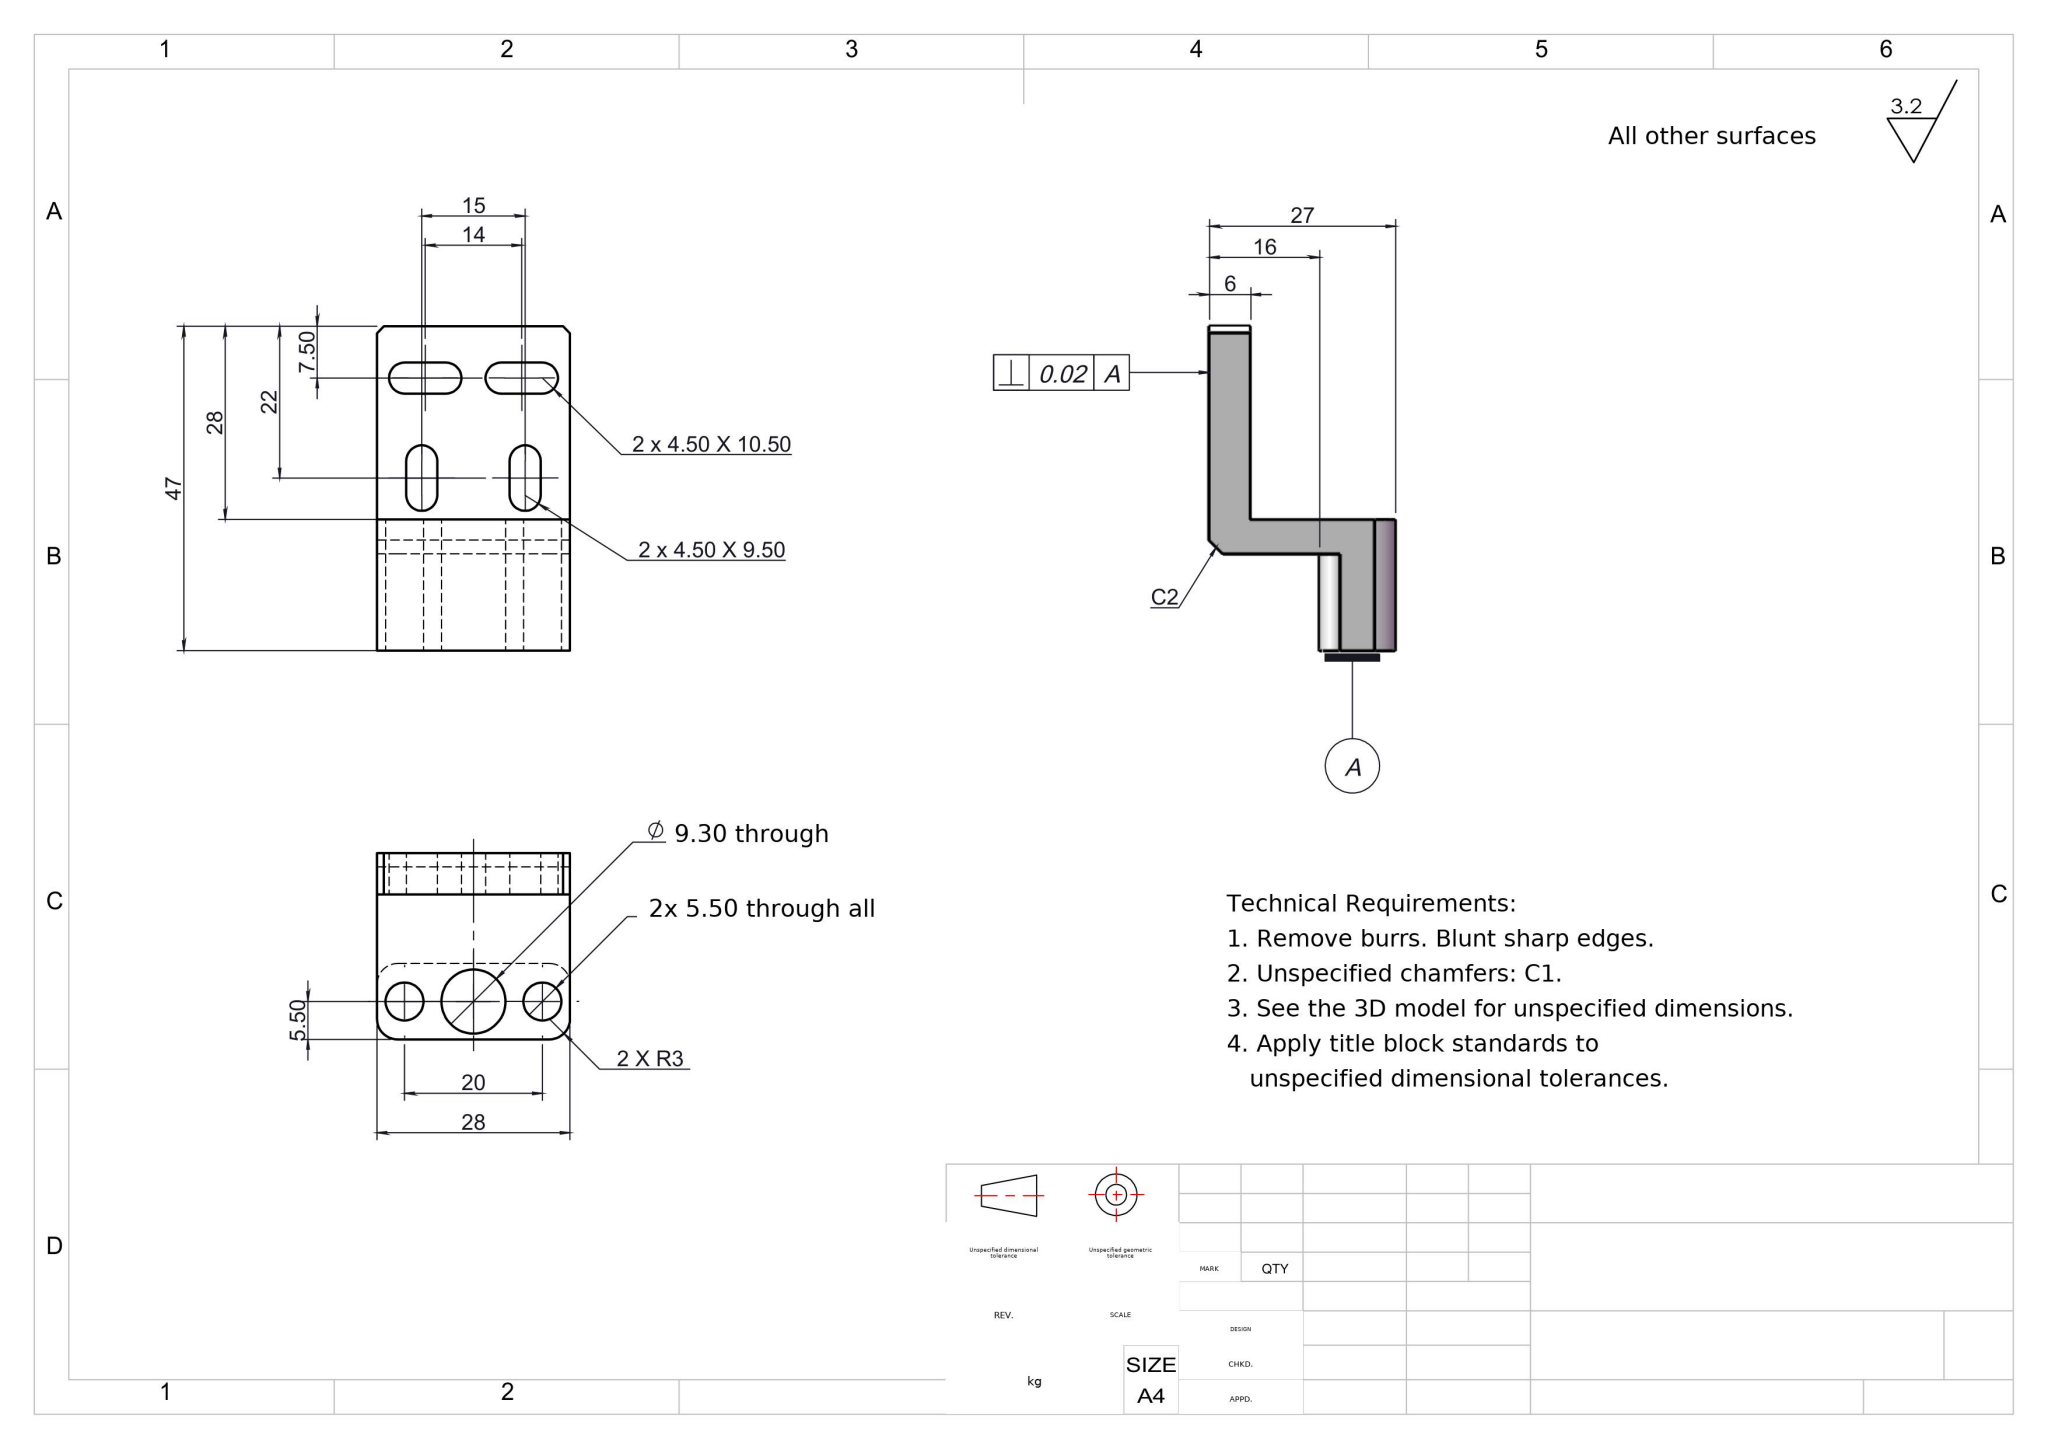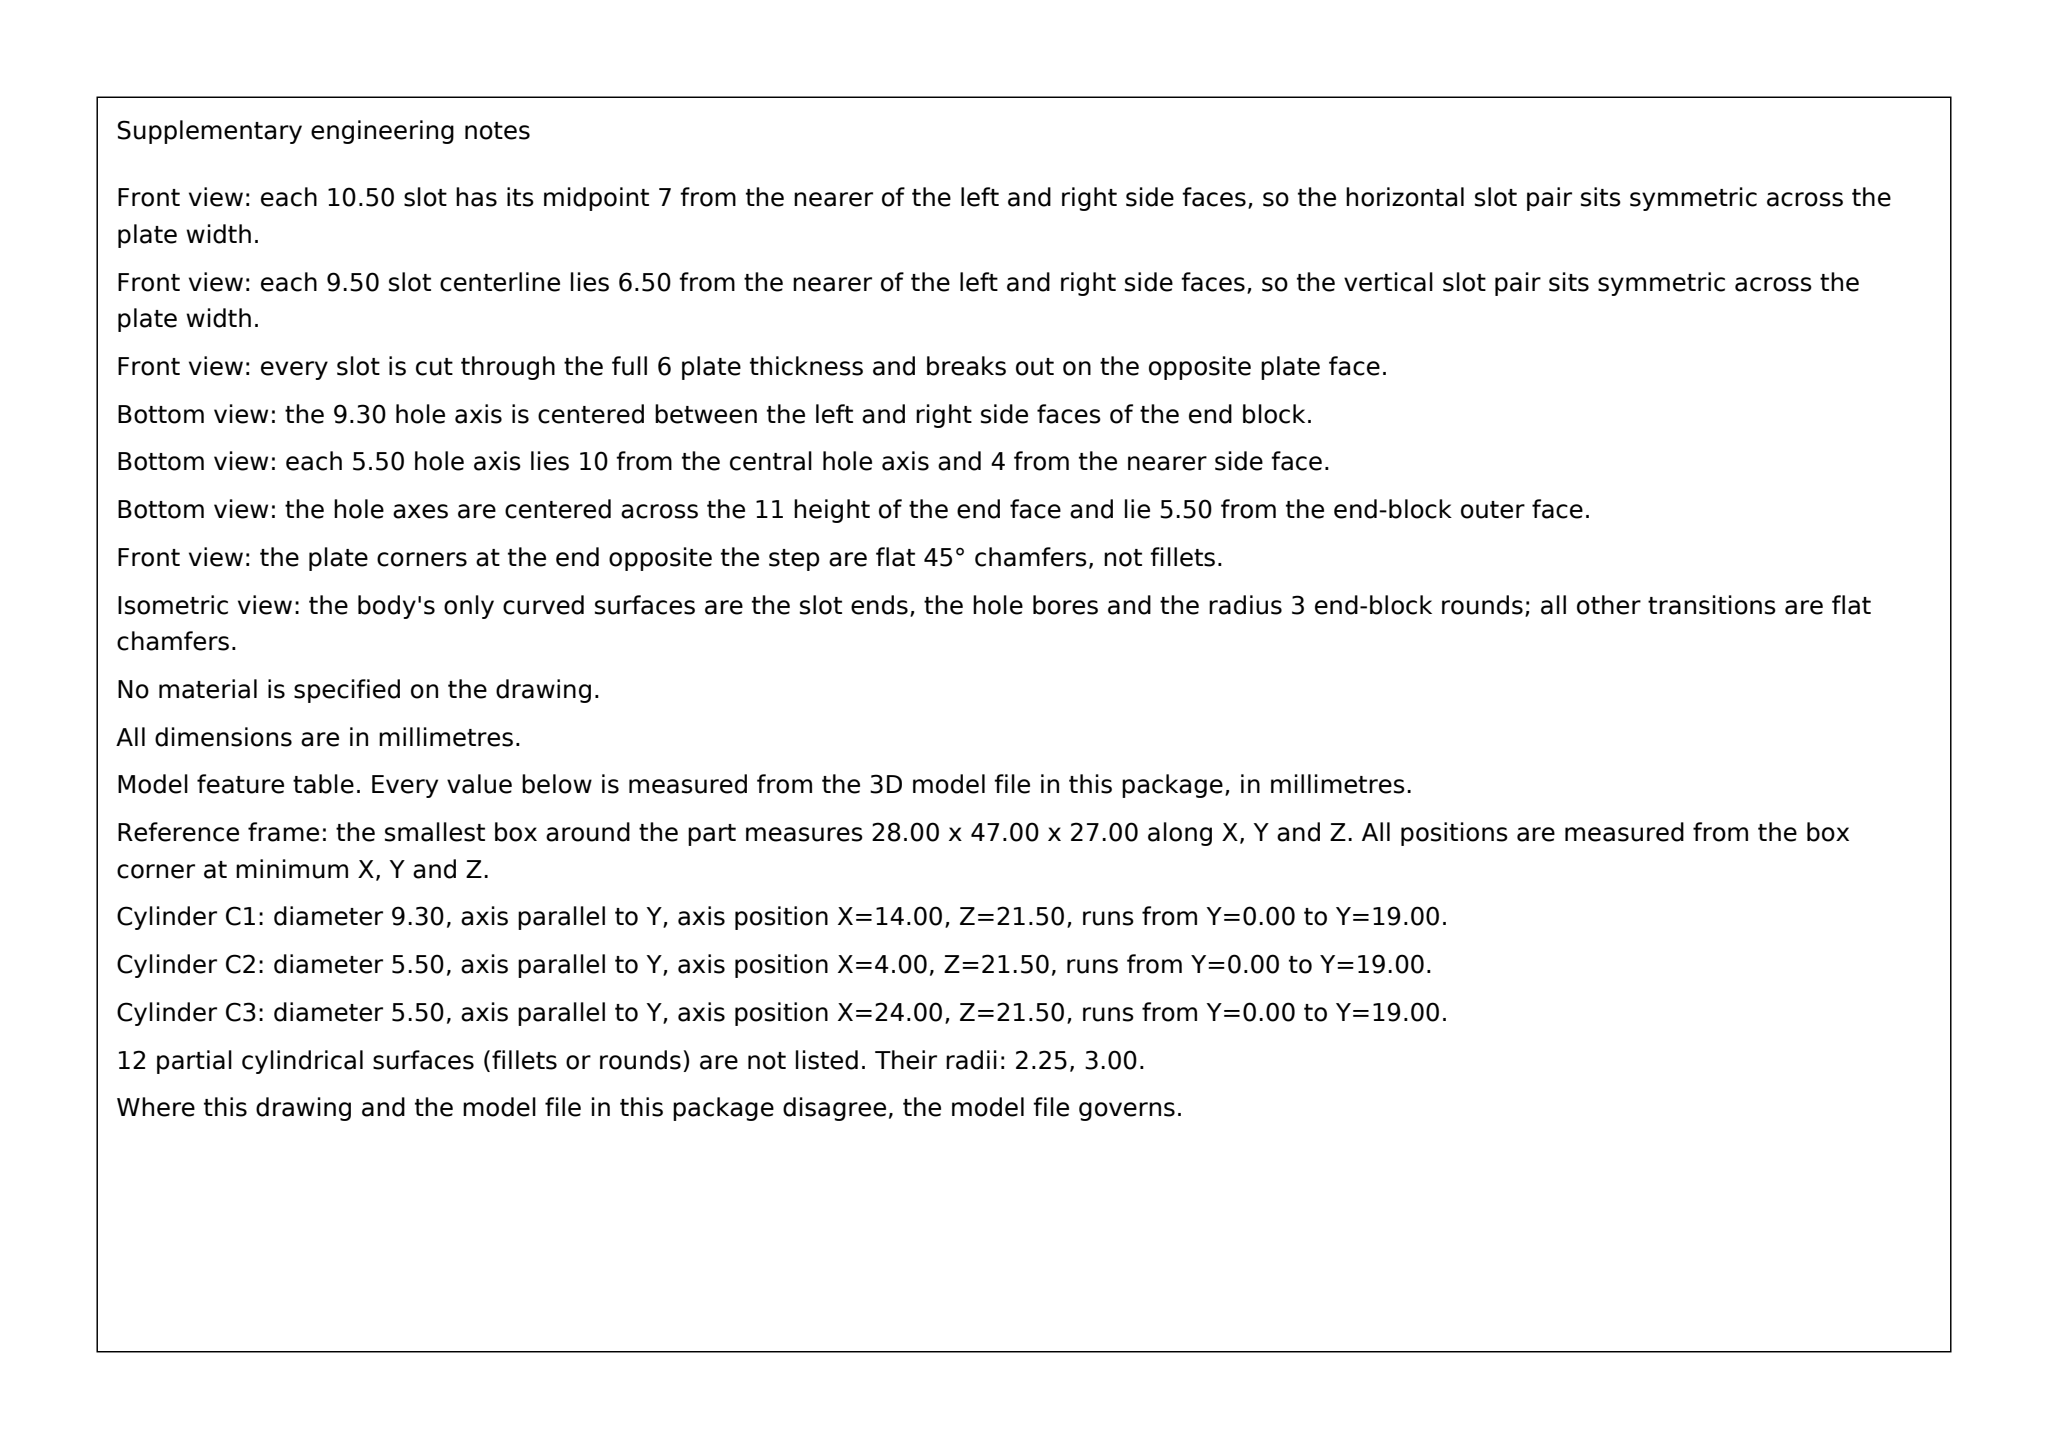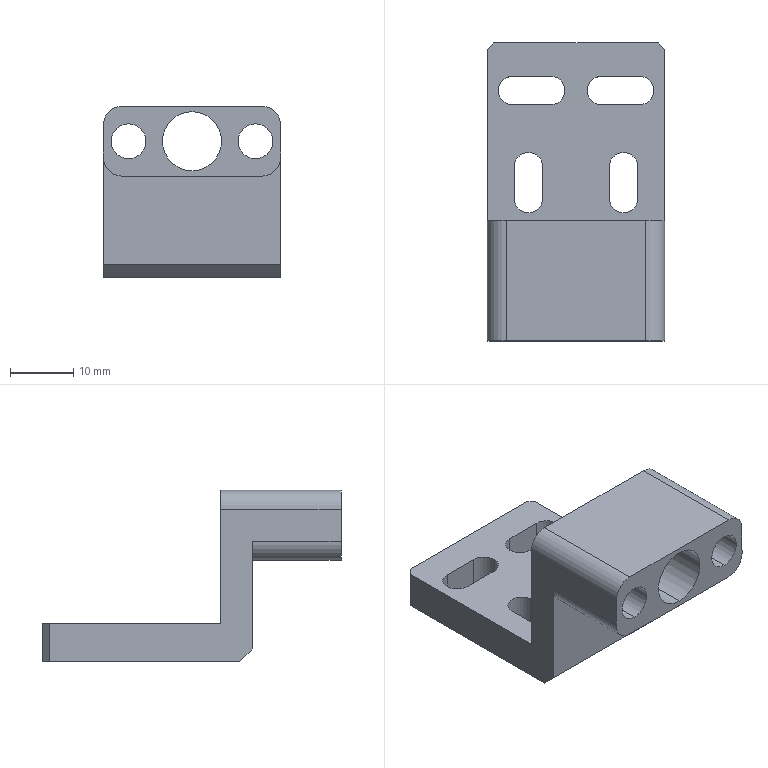Part | SolidWorks | mm | 1 solid | 41 faces | box 28 x 47 x 27 mm | volume 9437 mm3 | plane 21 | cylinder 20 | commonest cylinder face diameters 4.5 x10 5.5 x4 6 x4 9.3 x2
Drawing notes:
FOOT ARM 5 THK; END BLOCK 14 THK BELOW ARM, 19 TOTAL | from the solid: y planes 0/14/19: 19-14=5 arm, 14-0=14 block; Ø5.5 & Ø9.3 y-holes L=19
2 x 4.50 X 10.50 SLOTS: THRU ALL (6 PLATE) | from the solid: Ø4.5 z-axis cyls at y=39.5 (x=4,10,18,24), length 6.0 = full plate thickness z 0-6
2 x 4.50 X 9.50 SLOTS: THRU ALL (6 PLATE) | from the solid: Ø4.5 z-axis cyls at y=22.5/27.5 (x=6.5,21.5), length 6.0 = full plate thickness z 0-6